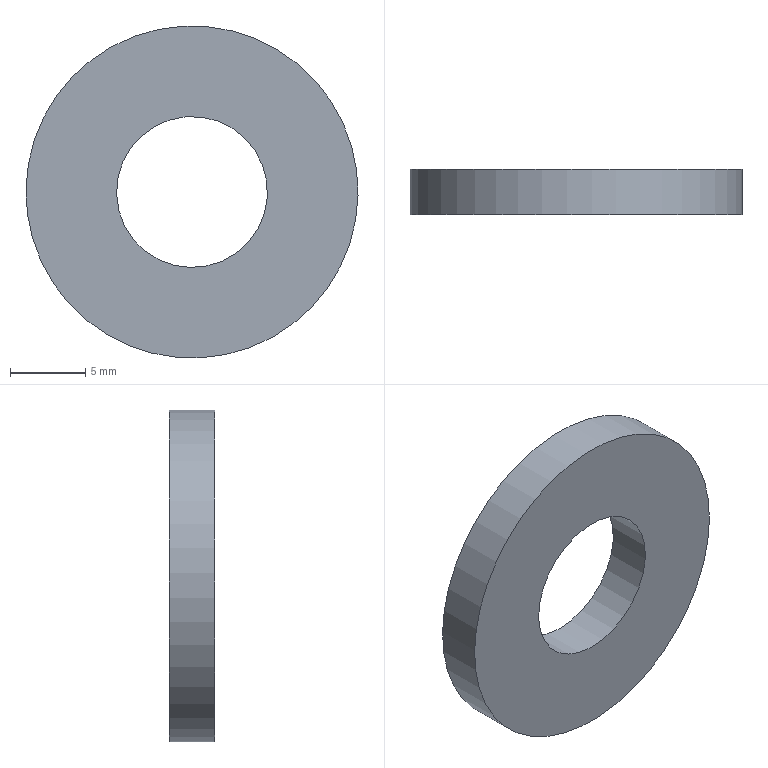Component | NX | JJZ-010 | 1 solid | 4 faces | box 22 x 3 x 22 mm | volume 905 mm3 | plane 2 | cylinder 2 | commonest cylinder face diameters 22 x1 10 x1
STEP:
#1=CARTESIAN_POINT('',(0.,0.,0.));
#2=DIRECTION('',(0.,0.,1.));
#3=DIRECTION('',(1.,0.,0.));
#4=AXIS2_PLACEMENT_3D('',#1,#2,#3);
#5=CARTESIAN_POINT('',(35.459,17.,-18.96));
#6=VERTEX_POINT('',#5);
#7=CARTESIAN_POINT('',(26.25,17.,-24.976));
#8=DIRECTION('',(0.,1.,0.));
#9=DIRECTION('',(0.8372,0.,0.5469));
#10=AXIS2_PLACEMENT_3D('',#7,#8,#9);
#11=CIRCLE('',#10,11.);
#12=CARTESIAN_POINT('',(26.25,17.,-24.976));
#13=DIRECTION('',(0.,-1.,0.));
#14=DIRECTION('',(-0.8372,0.,-0.5469));
#15=AXIS2_PLACEMENT_3D('',#12,#13,#14);
#16=PLANE('',#15);
#17=CARTESIAN_POINT('',(-11.,0.));
#18=CARTESIAN_POINT('',(-11.,19.053));
#19=CARTESIAN_POINT('',(5.5,9.526));
#20=CARTESIAN_POINT('',(22.,-0.));
#21=CARTESIAN_POINT('',(5.5,-9.526));
#22=CARTESIAN_POINT('',(-11.,-19.053));
#23=CARTESIAN_POINT('',(-11.,0.));
#24=(BOUNDED_CURVE()B_SPLINE_CURVE(2,(#17,#18,#19,#20,#21,#22,#23),.UNSPECIFIED.,.T.,.F.)B_SPLINE_CURVE_WITH_KNOTS((1,2,2,2,2,1),(-2.094,0.,2.094,4.189,6.283,8.378),.UNSPECIFIED.)CURVE()GEOMETRIC_REPRESENTATION_ITEM()RATIONAL_B_SPLINE_CURVE((1.,0.5,1.,0.5,1.,0.5,1.))REPRESENTATION_ITEM(''));
#25=(GEOMETRIC_REPRESENTATION_CONTEXT(2)PARAMETRIC_REPRESENTATION_CONTEXT()REPRESENTATION_CONTEXT('',''));
#26=DEFINITIONAL_REPRESENTATION('',(#24),#25);
#27=PCURVE('',#16,#26);
#28=CARTESIAN_POINT('',(26.25,17.,-24.976));
#29=DIRECTION('',(0.,1.,0.));
#30=DIRECTION('',(0.8372,0.,0.5469));
#31=AXIS2_PLACEMENT_3D('',#28,#29,#30);
#32=CYLINDRICAL_SURFACE('',#31,11.);
#33=CARTESIAN_POINT('',(0.,0.));
#34=DIRECTION('',(1.,0.));
#35=VECTOR('',#34,1.);
#36=LINE('',#33,#35);
#37=(GEOMETRIC_REPRESENTATION_CONTEXT(2)PARAMETRIC_REPRESENTATION_CONTEXT()REPRESENTATION_CONTEXT('',''));
#38=DEFINITIONAL_REPRESENTATION('',(#36),#37);
#39=PCURVE('',#32,#38);
#40=SURFACE_CURVE('',#11,(#27,#39),.PCURVE_S1.);
#41=EDGE_CURVE('',#6,#6,#40,.T.);
#42=ORIENTED_EDGE('',*,*,#41,.F.);
#43=EDGE_LOOP('',(#42));
#44=FACE_BOUND('',#43,.T.);
#45=CARTESIAN_POINT('',(30.436,17.,-22.241));
#46=VERTEX_POINT('',#45);
#47=CARTESIAN_POINT('',(26.25,17.,-24.976));
#48=DIRECTION('',(0.,1.,0.));
#49=DIRECTION('',(0.8372,0.,0.5469));
#50=AXIS2_PLACEMENT_3D('',#47,#48,#49);
#51=CIRCLE('',#50,5.);
#52=CARTESIAN_POINT('',(-5.,0.));
#53=CARTESIAN_POINT('',(-5.,8.66));
#54=CARTESIAN_POINT('',(2.5,4.33));
#55=CARTESIAN_POINT('',(10.,0.));
#56=CARTESIAN_POINT('',(2.5,-4.33));
#57=CARTESIAN_POINT('',(-5.,-8.66));
#58=CARTESIAN_POINT('',(-5.,0.));
#59=(BOUNDED_CURVE()B_SPLINE_CURVE(2,(#52,#53,#54,#55,#56,#57,#58),.UNSPECIFIED.,.T.,.F.)B_SPLINE_CURVE_WITH_KNOTS((1,2,2,2,2,1),(-2.094,0.,2.094,4.189,6.283,8.378),.UNSPECIFIED.)CURVE()GEOMETRIC_REPRESENTATION_ITEM()RATIONAL_B_SPLINE_CURVE((1.,0.5,1.,0.5,1.,0.5,1.))REPRESENTATION_ITEM(''));
#60=(GEOMETRIC_REPRESENTATION_CONTEXT(2)PARAMETRIC_REPRESENTATION_CONTEXT()REPRESENTATION_CONTEXT('',''));
#61=DEFINITIONAL_REPRESENTATION('',(#59),#60);
#62=PCURVE('',#16,#61);
#63=CARTESIAN_POINT('',(26.25,17.,-24.976));
#64=DIRECTION('',(0.,1.,0.));
#65=DIRECTION('',(0.8372,0.,0.5469));
#66=AXIS2_PLACEMENT_3D('',#63,#64,#65);
#67=CYLINDRICAL_SURFACE('',#66,5.);
#68=CARTESIAN_POINT('',(0.,0.));
#69=DIRECTION('',(1.,0.));
#70=VECTOR('',#69,1.);
#71=LINE('',#68,#70);
#72=(GEOMETRIC_REPRESENTATION_CONTEXT(2)PARAMETRIC_REPRESENTATION_CONTEXT()REPRESENTATION_CONTEXT('',''));
#73=DEFINITIONAL_REPRESENTATION('',(#71),#72);
#74=PCURVE('',#67,#73);
#75=SURFACE_CURVE('',#51,(#62,#74),.PCURVE_S1.);
#76=EDGE_CURVE('',#46,#46,#75,.T.);
#77=ORIENTED_EDGE('',*,*,#76,.T.);
#78=EDGE_LOOP('',(#77));
#79=FACE_BOUND('',#78,.T.);
#80=ADVANCED_FACE('',(#44,#79),#16,.T.);
#81=CARTESIAN_POINT('',(35.459,20.,-18.96));
#82=VERTEX_POINT('',#81);
#83=CARTESIAN_POINT('',(26.25,20.,-24.976));
#84=DIRECTION('',(0.,1.,0.));
#85=DIRECTION('',(0.8372,0.,0.5469));
#86=AXIS2_PLACEMENT_3D('',#83,#84,#85);
#87=CIRCLE('',#86,11.);
#88=CARTESIAN_POINT('',(26.25,20.,-24.976));
#89=DIRECTION('',(0.,-1.,0.));
#90=DIRECTION('',(-0.8372,0.,-0.5469));
#91=AXIS2_PLACEMENT_3D('',#88,#89,#90);
#92=PLANE('',#91);
#93=CARTESIAN_POINT('',(-11.,0.));
#94=CARTESIAN_POINT('',(-11.,19.053));
#95=CARTESIAN_POINT('',(5.5,9.526));
#96=CARTESIAN_POINT('',(22.,-0.));
#97=CARTESIAN_POINT('',(5.5,-9.526));
#98=CARTESIAN_POINT('',(-11.,-19.053));
#99=CARTESIAN_POINT('',(-11.,0.));
#100=(BOUNDED_CURVE()B_SPLINE_CURVE(2,(#93,#94,#95,#96,#97,#98,#99),.UNSPECIFIED.,.T.,.F.)B_SPLINE_CURVE_WITH_KNOTS((1,2,2,2,2,1),(-2.094,0.,2.094,4.189,6.283,8.378),.UNSPECIFIED.)CURVE()GEOMETRIC_REPRESENTATION_ITEM()RATIONAL_B_SPLINE_CURVE((1.,0.5,1.,0.5,1.,0.5,1.))REPRESENTATION_ITEM(''));
#101=(GEOMETRIC_REPRESENTATION_CONTEXT(2)PARAMETRIC_REPRESENTATION_CONTEXT()REPRESENTATION_CONTEXT('',''));
#102=DEFINITIONAL_REPRESENTATION('',(#100),#101);
#103=PCURVE('',#92,#102);
#104=CARTESIAN_POINT('',(0.,3.));
#105=DIRECTION('',(1.,0.));
#106=VECTOR('',#105,1.);
#107=LINE('',#104,#106);
#108=(GEOMETRIC_REPRESENTATION_CONTEXT(2)PARAMETRIC_REPRESENTATION_CONTEXT()REPRESENTATION_CONTEXT('',''));
#109=DEFINITIONAL_REPRESENTATION('',(#107),#108);
#110=PCURVE('',#32,#109);
#111=SURFACE_CURVE('',#87,(#103,#110),.PCURVE_S1.);
#112=EDGE_CURVE('',#82,#82,#111,.T.);
#113=ORIENTED_EDGE('',*,*,#112,.T.);
#114=EDGE_LOOP('',(#113));
#115=FACE_BOUND('',#114,.T.);
#116=CARTESIAN_POINT('',(30.436,20.,-22.241));
#117=VERTEX_POINT('',#116);
#118=CARTESIAN_POINT('',(26.25,20.,-24.976));
#119=DIRECTION('',(0.,1.,0.));
#120=DIRECTION('',(0.8372,0.,0.5469));
#121=AXIS2_PLACEMENT_3D('',#118,#119,#120);
#122=CIRCLE('',#121,5.);
#123=CARTESIAN_POINT('',(-5.,0.));
#124=CARTESIAN_POINT('',(-5.,8.66));
#125=CARTESIAN_POINT('',(2.5,4.33));
#126=CARTESIAN_POINT('',(10.,0.));
#127=CARTESIAN_POINT('',(2.5,-4.33));
#128=CARTESIAN_POINT('',(-5.,-8.66));
#129=CARTESIAN_POINT('',(-5.,0.));
#130=(BOUNDED_CURVE()B_SPLINE_CURVE(2,(#123,#124,#125,#126,#127,#128,#129),.UNSPECIFIED.,.T.,.F.)B_SPLINE_CURVE_WITH_KNOTS((1,2,2,2,2,1),(-2.094,0.,2.094,4.189,6.283,8.378),.UNSPECIFIED.)CURVE()GEOMETRIC_REPRESENTATION_ITEM()RATIONAL_B_SPLINE_CURVE((1.,0.5,1.,0.5,1.,0.5,1.))REPRESENTATION_ITEM(''));
#131=(GEOMETRIC_REPRESENTATION_CONTEXT(2)PARAMETRIC_REPRESENTATION_CONTEXT()REPRESENTATION_CONTEXT('',''));
#132=DEFINITIONAL_REPRESENTATION('',(#130),#131);
#133=PCURVE('',#92,#132);
#134=CARTESIAN_POINT('',(0.,3.));
#135=DIRECTION('',(1.,0.));
#136=VECTOR('',#135,1.);
#137=LINE('',#134,#136);
#138=(GEOMETRIC_REPRESENTATION_CONTEXT(2)PARAMETRIC_REPRESENTATION_CONTEXT()REPRESENTATION_CONTEXT('',''));
#139=DEFINITIONAL_REPRESENTATION('',(#137),#138);
#140=PCURVE('',#67,#139);
#141=SURFACE_CURVE('',#122,(#133,#140),.PCURVE_S1.);
#142=EDGE_CURVE('',#117,#117,#141,.T.);
#143=ORIENTED_EDGE('',*,*,#142,.F.);
#144=EDGE_LOOP('',(#143));
#145=FACE_BOUND('',#144,.T.);
#146=ADVANCED_FACE('',(#115,#145),#92,.F.);
#147=ORIENTED_EDGE('',*,*,#41,.T.);
#148=CARTESIAN_POINT('',(35.459,17.,-18.96));
#149=CARTESIAN_POINT('',(35.459,20.,-18.96));
#150=B_SPLINE_CURVE_WITH_KNOTS('',1,(#148,#149),.UNSPECIFIED.,.F.,.F.,(2,2),(0.,3.),.PIECEWISE_BEZIER_KNOTS.);
#151=CARTESIAN_POINT('',(6.283,0.));
#152=DIRECTION('',(0.,1.));
#153=VECTOR('',#152,1.);
#154=LINE('',#151,#153);
#155=(GEOMETRIC_REPRESENTATION_CONTEXT(2)PARAMETRIC_REPRESENTATION_CONTEXT()REPRESENTATION_CONTEXT('',''));
#156=DEFINITIONAL_REPRESENTATION('',(#154),#155);
#157=PCURVE('',#32,#156);
#158=CARTESIAN_POINT('',(0.,0.));
#159=DIRECTION('',(0.,1.));
#160=VECTOR('',#159,1.);
#161=LINE('',#158,#160);
#162=(GEOMETRIC_REPRESENTATION_CONTEXT(2)PARAMETRIC_REPRESENTATION_CONTEXT()REPRESENTATION_CONTEXT('',''));
#163=DEFINITIONAL_REPRESENTATION('',(#161),#162);
#164=PCURVE('',#32,#163);
#165=SEAM_CURVE('',#150,(#157,#164),.PCURVE_S1.);
#166=EDGE_CURVE('',#6,#82,#165,.T.);
#167=ORIENTED_EDGE('',*,*,#166,.T.);
#168=ORIENTED_EDGE('',*,*,#112,.F.);
#169=ORIENTED_EDGE('',*,*,#166,.F.);
#170=EDGE_LOOP('',(#147,#167,#168,#169));
#171=FACE_BOUND('',#170,.T.);
#172=ADVANCED_FACE('',(#171),#32,.T.);
#173=ORIENTED_EDGE('',*,*,#76,.T.);
#174=CARTESIAN_POINT('',(30.436,17.,-22.241));
#175=CARTESIAN_POINT('',(30.436,20.,-22.241));
#176=B_SPLINE_CURVE_WITH_KNOTS('',1,(#174,#175),.UNSPECIFIED.,.F.,.F.,(2,2),(0.,3.),.PIECEWISE_BEZIER_KNOTS.);
#177=CARTESIAN_POINT('',(6.283,0.));
#178=DIRECTION('',(0.,1.));
#179=VECTOR('',#178,1.);
#180=LINE('',#177,#179);
#181=(GEOMETRIC_REPRESENTATION_CONTEXT(2)PARAMETRIC_REPRESENTATION_CONTEXT()REPRESENTATION_CONTEXT('',''));
#182=DEFINITIONAL_REPRESENTATION('',(#180),#181);
#183=PCURVE('',#67,#182);
#184=CARTESIAN_POINT('',(0.,0.));
#185=DIRECTION('',(0.,1.));
#186=VECTOR('',#185,1.);
#187=LINE('',#184,#186);
#188=(GEOMETRIC_REPRESENTATION_CONTEXT(2)PARAMETRIC_REPRESENTATION_CONTEXT()REPRESENTATION_CONTEXT('',''));
#189=DEFINITIONAL_REPRESENTATION('',(#187),#188);
#190=PCURVE('',#67,#189);
#191=SEAM_CURVE('',#176,(#183,#190),.PCURVE_S1.);
#192=EDGE_CURVE('',#46,#117,#191,.T.);
#193=ORIENTED_EDGE('',*,*,#192,.T.);
#194=ORIENTED_EDGE('',*,*,#142,.F.);
#195=ORIENTED_EDGE('',*,*,#192,.F.);
#196=EDGE_LOOP('',(#173,#193,#194,#195));
#197=FACE_BOUND('',#196,.F.);
#198=ADVANCED_FACE('',(#197),#67,.F.);
#199=CLOSED_SHELL('',(#80,#146,#172,#198));
#200=MANIFOLD_SOLID_BREP('',#199);
#201=(LENGTH_UNIT()NAMED_UNIT(*)SI_UNIT(.MILLI.,.METRE.));
#202=UNCERTAINTY_MEASURE_WITH_UNIT(LENGTH_MEASURE(0.00001),#201,'','');
#203=(NAMED_UNIT(*)PLANE_ANGLE_UNIT()SI_UNIT($,.RADIAN.));
#204=(NAMED_UNIT(*)SI_UNIT($,.STERADIAN.)SOLID_ANGLE_UNIT());
#205=(GEOMETRIC_REPRESENTATION_CONTEXT(3)GLOBAL_UNCERTAINTY_ASSIGNED_CONTEXT((#202))GLOBAL_UNIT_ASSIGNED_CONTEXT((#201,#203,#204))REPRESENTATION_CONTEXT('',''));
#206=ADVANCED_BREP_SHAPE_REPRESENTATION('',(#4,#200),#205);